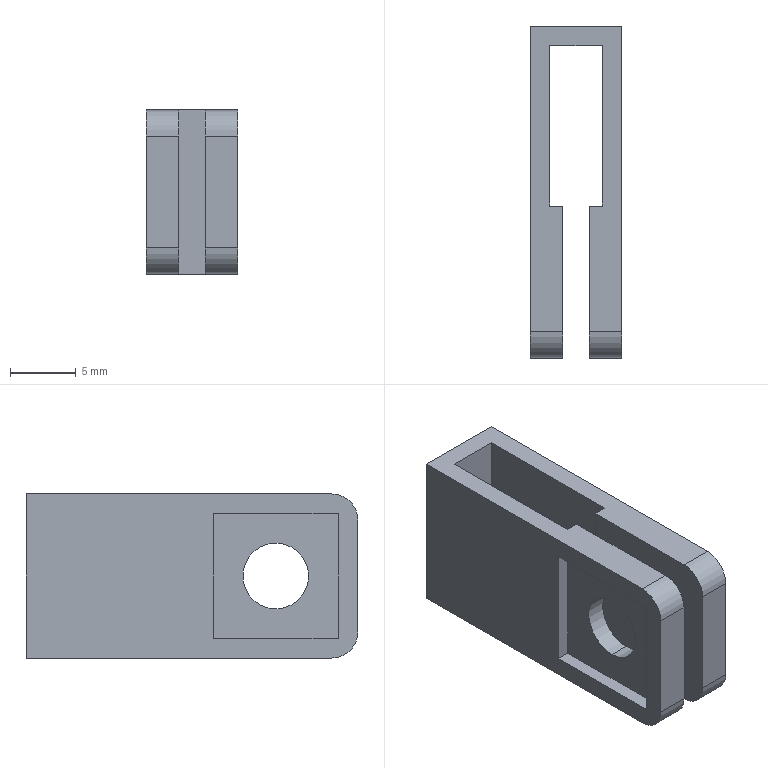Component | SolidWorks | GroundingSystem-1_CopperBarFixingClamp-1 | 1 solid | 32 faces | box 7 x 25.25 x 12.5 mm | volume 1063 mm3 | plane 24 | cylinder 8 | commonest cylinder face diameters 5 x4 4 x4
STEP:
#1=COLOUR_RGB('',0.7922,0.8196,0.9333);
#2=FILL_AREA_STYLE_COLOUR('',#1);
#3=FILL_AREA_STYLE('',(#2));
#4=SURFACE_STYLE_FILL_AREA(#3);
#5=SURFACE_SIDE_STYLE('',(#4));
#6=SURFACE_STYLE_USAGE(.BOTH.,#5);
#7=PRESENTATION_STYLE_ASSIGNMENT((#6));
#8=CARTESIAN_POINT('',(10.466,-0.8639,55.742));
#9=VERTEX_POINT('',#8);
#10=CARTESIAN_POINT('',(10.466,-0.8639,55.545));
#11=VERTEX_POINT('',#10);
#12=CARTESIAN_POINT('',(10.466,-0.8639,55.643));
#13=DIRECTION('',(-1.,0.,0.));
#14=DIRECTION('',(0.,-1.,0.));
#15=AXIS2_PLACEMENT_3D('',#12,#13,#14);
#16=CIRCLE('',#15,0.09843);
#17=EDGE_CURVE('',#9,#11,#16,.T.);
#18=ORIENTED_EDGE('',*,*,#17,.T.);
#19=CARTESIAN_POINT('',(10.525,-0.8639,55.545));
#20=VERTEX_POINT('',#19);
#21=CARTESIAN_POINT('',(10.289,-0.8639,55.545));
#22=DIRECTION('',(1.,-0.,-0.));
#23=VECTOR('',#22,39.37);
#24=LINE('',#21,#23);
#25=EDGE_CURVE('',#11,#20,#24,.T.);
#26=ORIENTED_EDGE('',*,*,#25,.T.);
#27=CARTESIAN_POINT('',(10.525,-0.8639,55.742));
#28=VERTEX_POINT('',#27);
#29=CARTESIAN_POINT('',(10.525,-0.8639,55.643));
#30=DIRECTION('',(-1.,0.,0.));
#31=DIRECTION('',(0.,0.,1.));
#32=AXIS2_PLACEMENT_3D('',#29,#30,#31);
#33=CIRCLE('',#32,0.09843);
#34=EDGE_CURVE('',#28,#20,#33,.T.);
#35=ORIENTED_EDGE('',*,*,#34,.F.);
#36=CARTESIAN_POINT('',(10.289,-0.8639,55.742));
#37=DIRECTION('',(1.,-0.,-0.));
#38=VECTOR('',#37,39.37);
#39=LINE('',#36,#38);
#40=EDGE_CURVE('',#9,#28,#39,.T.);
#41=ORIENTED_EDGE('',*,*,#40,.F.);
#42=EDGE_LOOP('',(#18,#26,#35,#41));
#43=FACE_OUTER_BOUND('',#42,.T.);
#44=CARTESIAN_POINT('',(10.289,-0.8639,55.643));
#45=DIRECTION('',(1.,-0.,-0.));
#46=DIRECTION('',(0.,0.,1.));
#47=AXIS2_PLACEMENT_3D('',#44,#45,#46);
#48=CYLINDRICAL_SURFACE('',#47,0.09843);
#49=ADVANCED_FACE('',(#43),#48,.F.);
#50=CARTESIAN_POINT('',(10.328,-0.8639,55.545));
#51=VERTEX_POINT('',#50);
#52=CARTESIAN_POINT('',(10.328,-0.8639,55.742));
#53=VERTEX_POINT('',#52);
#54=CARTESIAN_POINT('',(10.328,-0.8639,55.643));
#55=DIRECTION('',(1.,-0.,-0.));
#56=DIRECTION('',(0.,-0.,-1.));
#57=AXIS2_PLACEMENT_3D('',#54,#55,#56);
#58=CIRCLE('',#57,0.09843);
#59=EDGE_CURVE('',#51,#53,#58,.T.);
#60=ORIENTED_EDGE('',*,*,#59,.F.);
#61=CARTESIAN_POINT('',(10.387,-0.8639,55.545));
#62=VERTEX_POINT('',#61);
#63=CARTESIAN_POINT('',(10.289,-0.8639,55.545));
#64=DIRECTION('',(1.,-0.,-0.));
#65=VECTOR('',#64,39.37);
#66=LINE('',#63,#65);
#67=EDGE_CURVE('',#51,#62,#66,.T.);
#68=ORIENTED_EDGE('',*,*,#67,.T.);
#69=CARTESIAN_POINT('',(10.387,-0.8639,55.742));
#70=VERTEX_POINT('',#69);
#71=CARTESIAN_POINT('',(10.387,-0.8639,55.643));
#72=DIRECTION('',(1.,0.,-0.));
#73=DIRECTION('',(0.,1.,0.));
#74=AXIS2_PLACEMENT_3D('',#71,#72,#73);
#75=CIRCLE('',#74,0.09843);
#76=EDGE_CURVE('',#62,#70,#75,.T.);
#77=ORIENTED_EDGE('',*,*,#76,.T.);
#78=CARTESIAN_POINT('',(10.289,-0.8639,55.742));
#79=DIRECTION('',(1.,-0.,-0.));
#80=VECTOR('',#79,39.37);
#81=LINE('',#78,#80);
#82=EDGE_CURVE('',#53,#70,#81,.T.);
#83=ORIENTED_EDGE('',*,*,#82,.F.);
#84=EDGE_LOOP('',(#60,#68,#77,#83));
#85=FACE_OUTER_BOUND('',#84,.T.);
#86=CARTESIAN_POINT('',(10.289,-0.8639,55.643));
#87=DIRECTION('',(1.,-0.,-0.));
#88=DIRECTION('',(0.,0.,1.));
#89=AXIS2_PLACEMENT_3D('',#86,#87,#88);
#90=CYLINDRICAL_SURFACE('',#89,0.09843);
#91=ADVANCED_FACE('',(#85),#90,.F.);
#92=CARTESIAN_POINT('',(10.289,-0.1159,55.397));
#93=VERTEX_POINT('',#92);
#94=CARTESIAN_POINT('',(10.289,-1.031,55.397));
#95=VERTEX_POINT('',#94);
#96=CARTESIAN_POINT('',(10.289,-0.1159,55.397));
#97=DIRECTION('',(-0.,-1.,0.));
#98=VECTOR('',#97,39.37);
#99=LINE('',#96,#98);
#100=EDGE_CURVE('',#93,#95,#99,.T.);
#101=ORIENTED_EDGE('',*,*,#100,.T.);
#102=CARTESIAN_POINT('',(10.289,-1.11,55.476));
#103=VERTEX_POINT('',#102);
#104=CARTESIAN_POINT('',(10.289,-1.031,55.476));
#105=DIRECTION('',(-1.,0.,0.));
#106=DIRECTION('',(0.,-0.,-1.));
#107=AXIS2_PLACEMENT_3D('',#104,#105,#106);
#108=CIRCLE('',#107,0.07874);
#109=EDGE_CURVE('',#95,#103,#108,.T.);
#110=ORIENTED_EDGE('',*,*,#109,.T.);
#111=CARTESIAN_POINT('',(10.289,-1.11,55.811));
#112=VERTEX_POINT('',#111);
#113=CARTESIAN_POINT('',(10.289,-1.11,55.397));
#114=DIRECTION('',(0.,0.,1.));
#115=VECTOR('',#114,39.37);
#116=LINE('',#113,#115);
#117=EDGE_CURVE('',#103,#112,#116,.T.);
#118=ORIENTED_EDGE('',*,*,#117,.T.);
#119=CARTESIAN_POINT('',(10.289,-1.031,55.889));
#120=VERTEX_POINT('',#119);
#121=CARTESIAN_POINT('',(10.289,-1.031,55.811));
#122=DIRECTION('',(-1.,0.,0.));
#123=DIRECTION('',(0.,-0.,-1.));
#124=AXIS2_PLACEMENT_3D('',#121,#122,#123);
#125=CIRCLE('',#124,0.07874);
#126=EDGE_CURVE('',#112,#120,#125,.T.);
#127=ORIENTED_EDGE('',*,*,#126,.T.);
#128=CARTESIAN_POINT('',(10.289,-0.1159,55.889));
#129=VERTEX_POINT('',#128);
#130=CARTESIAN_POINT('',(10.289,-0.1159,55.889));
#131=DIRECTION('',(-0.,-1.,0.));
#132=VECTOR('',#131,39.37);
#133=LINE('',#130,#132);
#134=EDGE_CURVE('',#129,#120,#133,.T.);
#135=ORIENTED_EDGE('',*,*,#134,.F.);
#136=CARTESIAN_POINT('',(10.289,-0.1159,55.397));
#137=DIRECTION('',(0.,0.,1.));
#138=VECTOR('',#137,39.37);
#139=LINE('',#136,#138);
#140=EDGE_CURVE('',#93,#129,#139,.T.);
#141=ORIENTED_EDGE('',*,*,#140,.F.);
#142=EDGE_LOOP('',(#101,#110,#118,#127,#135,#141));
#143=FACE_OUTER_BOUND('',#142,.T.);
#144=CARTESIAN_POINT('',(10.289,-0.6769,55.83));
#145=VERTEX_POINT('',#144);
#146=CARTESIAN_POINT('',(10.289,-1.051,55.83));
#147=VERTEX_POINT('',#146);
#148=CARTESIAN_POINT('',(10.289,-0.6769,55.83));
#149=DIRECTION('',(-0.,-1.,0.));
#150=VECTOR('',#149,39.37);
#151=LINE('',#148,#150);
#152=EDGE_CURVE('',#145,#147,#151,.T.);
#153=ORIENTED_EDGE('',*,*,#152,.T.);
#154=CARTESIAN_POINT('',(10.289,-1.051,55.456));
#155=VERTEX_POINT('',#154);
#156=CARTESIAN_POINT('',(10.289,-1.051,55.83));
#157=DIRECTION('',(-0.,-0.,-1.));
#158=VECTOR('',#157,39.37);
#159=LINE('',#156,#158);
#160=EDGE_CURVE('',#147,#155,#159,.T.);
#161=ORIENTED_EDGE('',*,*,#160,.T.);
#162=CARTESIAN_POINT('',(10.289,-0.6769,55.456));
#163=VERTEX_POINT('',#162);
#164=CARTESIAN_POINT('',(10.289,-1.051,55.456));
#165=DIRECTION('',(0.,1.,-0.));
#166=VECTOR('',#165,39.37);
#167=LINE('',#164,#166);
#168=EDGE_CURVE('',#155,#163,#167,.T.);
#169=ORIENTED_EDGE('',*,*,#168,.T.);
#170=CARTESIAN_POINT('',(10.289,-0.6769,55.456));
#171=DIRECTION('',(0.,0.,1.));
#172=VECTOR('',#171,39.37);
#173=LINE('',#170,#172);
#174=EDGE_CURVE('',#163,#145,#173,.T.);
#175=ORIENTED_EDGE('',*,*,#174,.T.);
#176=EDGE_LOOP('',(#153,#161,#169,#175));
#177=FACE_BOUND('',#176,.T.);
#178=CARTESIAN_POINT('',(10.289,-0.1159,55.397));
#179=DIRECTION('',(-1.,0.,0.));
#180=DIRECTION('',(-0.,-0.,-1.));
#181=AXIS2_PLACEMENT_3D('',#178,#179,#180);
#182=PLANE('',#181);
#183=ADVANCED_FACE('',(#143,#177),#182,.T.);
#184=ORIENTED_EDGE('',*,*,#67,.F.);
#185=CARTESIAN_POINT('',(10.328,-0.8639,55.643));
#186=DIRECTION('',(1.,-0.,-0.));
#187=DIRECTION('',(0.,-0.,-1.));
#188=AXIS2_PLACEMENT_3D('',#185,#186,#187);
#189=CIRCLE('',#188,0.09843);
#190=EDGE_CURVE('',#53,#51,#189,.T.);
#191=ORIENTED_EDGE('',*,*,#190,.F.);
#192=ORIENTED_EDGE('',*,*,#82,.T.);
#193=CARTESIAN_POINT('',(10.387,-0.8639,55.643));
#194=DIRECTION('',(1.,0.,-0.));
#195=DIRECTION('',(0.,1.,0.));
#196=AXIS2_PLACEMENT_3D('',#193,#194,#195);
#197=CIRCLE('',#196,0.09843);
#198=EDGE_CURVE('',#70,#62,#197,.T.);
#199=ORIENTED_EDGE('',*,*,#198,.T.);
#200=EDGE_LOOP('',(#184,#191,#192,#199));
#201=FACE_OUTER_BOUND('',#200,.T.);
#202=CARTESIAN_POINT('',(10.289,-0.8639,55.643));
#203=DIRECTION('',(1.,-0.,-0.));
#204=DIRECTION('',(0.,0.,1.));
#205=AXIS2_PLACEMENT_3D('',#202,#203,#204);
#206=CYLINDRICAL_SURFACE('',#205,0.09843);
#207=ADVANCED_FACE('',(#201),#206,.F.);
#208=ORIENTED_EDGE('',*,*,#25,.F.);
#209=CARTESIAN_POINT('',(10.466,-0.8639,55.643));
#210=DIRECTION('',(-1.,0.,0.));
#211=DIRECTION('',(0.,-1.,0.));
#212=AXIS2_PLACEMENT_3D('',#209,#210,#211);
#213=CIRCLE('',#212,0.09843);
#214=EDGE_CURVE('',#11,#9,#213,.T.);
#215=ORIENTED_EDGE('',*,*,#214,.T.);
#216=ORIENTED_EDGE('',*,*,#40,.T.);
#217=CARTESIAN_POINT('',(10.525,-0.8639,55.643));
#218=DIRECTION('',(-1.,0.,0.));
#219=DIRECTION('',(0.,0.,1.));
#220=AXIS2_PLACEMENT_3D('',#217,#218,#219);
#221=CIRCLE('',#220,0.09843);
#222=EDGE_CURVE('',#20,#28,#221,.T.);
#223=ORIENTED_EDGE('',*,*,#222,.F.);
#224=EDGE_LOOP('',(#208,#215,#216,#223));
#225=FACE_OUTER_BOUND('',#224,.T.);
#226=CARTESIAN_POINT('',(10.289,-0.8639,55.643));
#227=DIRECTION('',(1.,-0.,-0.));
#228=DIRECTION('',(0.,0.,1.));
#229=AXIS2_PLACEMENT_3D('',#226,#227,#228);
#230=CYLINDRICAL_SURFACE('',#229,0.09843);
#231=ADVANCED_FACE('',(#225),#230,.F.);
#232=CARTESIAN_POINT('',(10.466,-1.11,55.811));
#233=VERTEX_POINT('',#232);
#234=CARTESIAN_POINT('',(10.466,-1.11,55.476));
#235=VERTEX_POINT('',#234);
#236=CARTESIAN_POINT('',(10.466,-1.11,55.397));
#237=DIRECTION('',(-0.,-0.,-1.));
#238=VECTOR('',#237,39.37);
#239=LINE('',#236,#238);
#240=EDGE_CURVE('',#233,#235,#239,.T.);
#241=ORIENTED_EDGE('',*,*,#240,.T.);
#242=CARTESIAN_POINT('',(10.564,-1.11,55.476));
#243=VERTEX_POINT('',#242);
#244=CARTESIAN_POINT('',(10.289,-1.11,55.476));
#245=DIRECTION('',(1.,-0.,-0.));
#246=VECTOR('',#245,39.37);
#247=LINE('',#244,#246);
#248=EDGE_CURVE('',#235,#243,#247,.T.);
#249=ORIENTED_EDGE('',*,*,#248,.T.);
#250=CARTESIAN_POINT('',(10.564,-1.11,55.811));
#251=VERTEX_POINT('',#250);
#252=CARTESIAN_POINT('',(10.564,-1.11,55.397));
#253=DIRECTION('',(0.,0.,1.));
#254=VECTOR('',#253,39.37);
#255=LINE('',#252,#254);
#256=EDGE_CURVE('',#243,#251,#255,.T.);
#257=ORIENTED_EDGE('',*,*,#256,.T.);
#258=CARTESIAN_POINT('',(10.466,-1.11,55.811));
#259=DIRECTION('',(-1.,0.,0.));
#260=VECTOR('',#259,39.37);
#261=LINE('',#258,#260);
#262=EDGE_CURVE('',#251,#233,#261,.T.);
#263=ORIENTED_EDGE('',*,*,#262,.T.);
#264=EDGE_LOOP('',(#241,#249,#257,#263));
#265=FACE_OUTER_BOUND('',#264,.T.);
#266=CARTESIAN_POINT('',(10.289,-1.11,55.397));
#267=DIRECTION('',(-0.,-1.,0.));
#268=DIRECTION('',(-0.,-0.,-1.));
#269=AXIS2_PLACEMENT_3D('',#266,#267,#268);
#270=PLANE('',#269);
#271=ADVANCED_FACE('',(#265),#270,.T.);
#272=ORIENTED_EDGE('',*,*,#117,.F.);
#273=CARTESIAN_POINT('',(10.387,-1.11,55.476));
#274=VERTEX_POINT('',#273);
#275=CARTESIAN_POINT('',(10.289,-1.11,55.476));
#276=DIRECTION('',(1.,-0.,-0.));
#277=VECTOR('',#276,39.37);
#278=LINE('',#275,#277);
#279=EDGE_CURVE('',#103,#274,#278,.T.);
#280=ORIENTED_EDGE('',*,*,#279,.T.);
#281=CARTESIAN_POINT('',(10.387,-1.11,55.811));
#282=VERTEX_POINT('',#281);
#283=CARTESIAN_POINT('',(10.387,-1.11,55.397));
#284=DIRECTION('',(0.,0.,1.));
#285=VECTOR('',#284,39.37);
#286=LINE('',#283,#285);
#287=EDGE_CURVE('',#274,#282,#286,.T.);
#288=ORIENTED_EDGE('',*,*,#287,.T.);
#289=CARTESIAN_POINT('',(10.289,-1.11,55.811));
#290=DIRECTION('',(-1.,0.,0.));
#291=VECTOR('',#290,39.37);
#292=LINE('',#289,#291);
#293=EDGE_CURVE('',#282,#112,#292,.T.);
#294=ORIENTED_EDGE('',*,*,#293,.T.);
#295=EDGE_LOOP('',(#272,#280,#288,#294));
#296=FACE_OUTER_BOUND('',#295,.T.);
#297=CARTESIAN_POINT('',(10.289,-1.11,55.397));
#298=DIRECTION('',(-0.,-1.,0.));
#299=DIRECTION('',(-0.,-0.,-1.));
#300=AXIS2_PLACEMENT_3D('',#297,#298,#299);
#301=PLANE('',#300);
#302=ADVANCED_FACE('',(#296),#301,.T.);
#303=CARTESIAN_POINT('',(10.387,-0.6553,55.397));
#304=VERTEX_POINT('',#303);
#305=CARTESIAN_POINT('',(10.387,-1.031,55.397));
#306=VERTEX_POINT('',#305);
#307=CARTESIAN_POINT('',(10.387,-1.11,55.397));
#308=DIRECTION('',(0.,-1.,0.));
#309=VECTOR('',#308,39.37);
#310=LINE('',#307,#309);
#311=EDGE_CURVE('',#304,#306,#310,.T.);
#312=ORIENTED_EDGE('',*,*,#311,.T.);
#313=CARTESIAN_POINT('',(10.564,-1.031,55.397));
#314=DIRECTION('',(-1.,0.,0.));
#315=VECTOR('',#314,39.37);
#316=LINE('',#313,#315);
#317=EDGE_CURVE('',#306,#95,#316,.T.);
#318=ORIENTED_EDGE('',*,*,#317,.T.);
#319=ORIENTED_EDGE('',*,*,#100,.F.);
#320=CARTESIAN_POINT('',(10.564,-0.1159,55.397));
#321=VERTEX_POINT('',#320);
#322=CARTESIAN_POINT('',(10.289,-0.1159,55.397));
#323=DIRECTION('',(-1.,0.,0.));
#324=VECTOR('',#323,39.37);
#325=LINE('',#322,#324);
#326=EDGE_CURVE('',#321,#93,#325,.T.);
#327=ORIENTED_EDGE('',*,*,#326,.F.);
#328=CARTESIAN_POINT('',(10.564,-1.031,55.397));
#329=VERTEX_POINT('',#328);
#330=CARTESIAN_POINT('',(10.564,-0.1159,55.397));
#331=DIRECTION('',(0.,1.,-0.));
#332=VECTOR('',#331,39.37);
#333=LINE('',#330,#332);
#334=EDGE_CURVE('',#329,#321,#333,.T.);
#335=ORIENTED_EDGE('',*,*,#334,.F.);
#336=CARTESIAN_POINT('',(10.466,-1.031,55.397));
#337=VERTEX_POINT('',#336);
#338=CARTESIAN_POINT('',(10.564,-1.031,55.397));
#339=DIRECTION('',(-1.,0.,0.));
#340=VECTOR('',#339,39.37);
#341=LINE('',#338,#340);
#342=EDGE_CURVE('',#329,#337,#341,.T.);
#343=ORIENTED_EDGE('',*,*,#342,.T.);
#344=CARTESIAN_POINT('',(10.466,-0.6553,55.397));
#345=VERTEX_POINT('',#344);
#346=CARTESIAN_POINT('',(10.466,-1.11,55.397));
#347=DIRECTION('',(0.,1.,-0.));
#348=VECTOR('',#347,39.37);
#349=LINE('',#346,#348);
#350=EDGE_CURVE('',#337,#345,#349,.T.);
#351=ORIENTED_EDGE('',*,*,#350,.T.);
#352=CARTESIAN_POINT('',(10.505,-0.6553,55.397));
#353=VERTEX_POINT('',#352);
#354=CARTESIAN_POINT('',(10.564,-0.6553,55.397));
#355=DIRECTION('',(1.,-0.,-0.));
#356=VECTOR('',#355,39.37);
#357=LINE('',#354,#356);
#358=EDGE_CURVE('',#345,#353,#357,.T.);
#359=ORIENTED_EDGE('',*,*,#358,.T.);
#360=CARTESIAN_POINT('',(10.505,-0.175,55.397));
#361=VERTEX_POINT('',#360);
#362=CARTESIAN_POINT('',(10.505,-1.11,55.397));
#363=DIRECTION('',(0.,1.,-0.));
#364=VECTOR('',#363,39.37);
#365=LINE('',#362,#364);
#366=EDGE_CURVE('',#353,#361,#365,.T.);
#367=ORIENTED_EDGE('',*,*,#366,.T.);
#368=CARTESIAN_POINT('',(10.348,-0.175,55.397));
#369=VERTEX_POINT('',#368);
#370=CARTESIAN_POINT('',(10.564,-0.175,55.397));
#371=DIRECTION('',(-1.,0.,0.));
#372=VECTOR('',#371,39.37);
#373=LINE('',#370,#372);
#374=EDGE_CURVE('',#361,#369,#373,.T.);
#375=ORIENTED_EDGE('',*,*,#374,.T.);
#376=CARTESIAN_POINT('',(10.348,-0.6553,55.397));
#377=VERTEX_POINT('',#376);
#378=CARTESIAN_POINT('',(10.348,-1.11,55.397));
#379=DIRECTION('',(0.,-1.,0.));
#380=VECTOR('',#379,39.37);
#381=LINE('',#378,#380);
#382=EDGE_CURVE('',#369,#377,#381,.T.);
#383=ORIENTED_EDGE('',*,*,#382,.T.);
#384=CARTESIAN_POINT('',(10.564,-0.6553,55.397));
#385=DIRECTION('',(1.,0.,-0.));
#386=VECTOR('',#385,39.37);
#387=LINE('',#384,#386);
#388=EDGE_CURVE('',#377,#304,#387,.T.);
#389=ORIENTED_EDGE('',*,*,#388,.T.);
#390=EDGE_LOOP('',(#312,#318,#319,#327,#335,#343,#351,#359,#367,#375,#383,#389));
#391=FACE_OUTER_BOUND('',#390,.T.);
#392=CARTESIAN_POINT('',(10.564,-1.11,55.397));
#393=DIRECTION('',(-0.,-0.,-1.));
#394=DIRECTION('',(0.,1.,-0.));
#395=AXIS2_PLACEMENT_3D('',#392,#393,#394);
#396=PLANE('',#395);
#397=ADVANCED_FACE('',(#391),#396,.T.);
#398=CARTESIAN_POINT('',(10.466,-1.031,55.889));
#399=VERTEX_POINT('',#398);
#400=CARTESIAN_POINT('',(10.466,-0.6553,55.889));
#401=VERTEX_POINT('',#400);
#402=CARTESIAN_POINT('',(10.466,-1.11,55.889));
#403=DIRECTION('',(0.,1.,-0.));
#404=VECTOR('',#403,39.37);
#405=LINE('',#402,#404);
#406=EDGE_CURVE('',#399,#401,#405,.T.);
#407=ORIENTED_EDGE('',*,*,#406,.F.);
#408=CARTESIAN_POINT('',(10.564,-1.031,55.889));
#409=VERTEX_POINT('',#408);
#410=CARTESIAN_POINT('',(10.564,-1.031,55.889));
#411=DIRECTION('',(1.,-0.,-0.));
#412=VECTOR('',#411,39.37);
#413=LINE('',#410,#412);
#414=EDGE_CURVE('',#399,#409,#413,.T.);
#415=ORIENTED_EDGE('',*,*,#414,.T.);
#416=CARTESIAN_POINT('',(10.564,-0.1159,55.889));
#417=VERTEX_POINT('',#416);
#418=CARTESIAN_POINT('',(10.564,-0.1159,55.889));
#419=DIRECTION('',(0.,1.,-0.));
#420=VECTOR('',#419,39.37);
#421=LINE('',#418,#420);
#422=EDGE_CURVE('',#409,#417,#421,.T.);
#423=ORIENTED_EDGE('',*,*,#422,.T.);
#424=CARTESIAN_POINT('',(10.289,-0.1159,55.889));
#425=DIRECTION('',(-1.,0.,0.));
#426=VECTOR('',#425,39.37);
#427=LINE('',#424,#426);
#428=EDGE_CURVE('',#417,#129,#427,.T.);
#429=ORIENTED_EDGE('',*,*,#428,.T.);
#430=ORIENTED_EDGE('',*,*,#134,.T.);
#431=CARTESIAN_POINT('',(10.387,-1.031,55.889));
#432=VERTEX_POINT('',#431);
#433=CARTESIAN_POINT('',(10.387,-1.031,55.889));
#434=DIRECTION('',(1.,-0.,-0.));
#435=VECTOR('',#434,39.37);
#436=LINE('',#433,#435);
#437=EDGE_CURVE('',#120,#432,#436,.T.);
#438=ORIENTED_EDGE('',*,*,#437,.T.);
#439=CARTESIAN_POINT('',(10.387,-0.6553,55.889));
#440=VERTEX_POINT('',#439);
#441=CARTESIAN_POINT('',(10.387,-1.11,55.889));
#442=DIRECTION('',(0.,-1.,0.));
#443=VECTOR('',#442,39.37);
#444=LINE('',#441,#443);
#445=EDGE_CURVE('',#440,#432,#444,.T.);
#446=ORIENTED_EDGE('',*,*,#445,.F.);
#447=CARTESIAN_POINT('',(10.348,-0.6553,55.889));
#448=VERTEX_POINT('',#447);
#449=CARTESIAN_POINT('',(10.564,-0.6553,55.889));
#450=DIRECTION('',(1.,0.,-0.));
#451=VECTOR('',#450,39.37);
#452=LINE('',#449,#451);
#453=EDGE_CURVE('',#448,#440,#452,.T.);
#454=ORIENTED_EDGE('',*,*,#453,.F.);
#455=CARTESIAN_POINT('',(10.348,-0.175,55.889));
#456=VERTEX_POINT('',#455);
#457=CARTESIAN_POINT('',(10.348,-1.11,55.889));
#458=DIRECTION('',(0.,-1.,0.));
#459=VECTOR('',#458,39.37);
#460=LINE('',#457,#459);
#461=EDGE_CURVE('',#456,#448,#460,.T.);
#462=ORIENTED_EDGE('',*,*,#461,.F.);
#463=CARTESIAN_POINT('',(10.505,-0.175,55.889));
#464=VERTEX_POINT('',#463);
#465=CARTESIAN_POINT('',(10.564,-0.175,55.889));
#466=DIRECTION('',(-1.,0.,0.));
#467=VECTOR('',#466,39.37);
#468=LINE('',#465,#467);
#469=EDGE_CURVE('',#464,#456,#468,.T.);
#470=ORIENTED_EDGE('',*,*,#469,.F.);
#471=CARTESIAN_POINT('',(10.505,-0.6553,55.889));
#472=VERTEX_POINT('',#471);
#473=CARTESIAN_POINT('',(10.505,-1.11,55.889));
#474=DIRECTION('',(0.,1.,-0.));
#475=VECTOR('',#474,39.37);
#476=LINE('',#473,#475);
#477=EDGE_CURVE('',#472,#464,#476,.T.);
#478=ORIENTED_EDGE('',*,*,#477,.F.);
#479=CARTESIAN_POINT('',(10.564,-0.6553,55.889));
#480=DIRECTION('',(1.,-0.,-0.));
#481=VECTOR('',#480,39.37);
#482=LINE('',#479,#481);
#483=EDGE_CURVE('',#401,#472,#482,.T.);
#484=ORIENTED_EDGE('',*,*,#483,.F.);
#485=EDGE_LOOP('',(#407,#415,#423,#429,#430,#438,#446,#454,#462,#470,#478,#484));
#486=FACE_OUTER_BOUND('',#485,.T.);
#487=CARTESIAN_POINT('',(10.564,-1.11,55.889));
#488=DIRECTION('',(-0.,-0.,-1.));
#489=DIRECTION('',(0.,1.,-0.));
#490=AXIS2_PLACEMENT_3D('',#487,#488,#489);
#491=PLANE('',#490);
#492=ADVANCED_FACE('',(#486),#491,.F.);
#493=ORIENTED_EDGE('',*,*,#428,.F.);
#494=CARTESIAN_POINT('',(10.564,-0.1159,55.397));
#495=DIRECTION('',(0.,0.,1.));
#496=VECTOR('',#495,39.37);
#497=LINE('',#494,#496);
#498=EDGE_CURVE('',#321,#417,#497,.T.);
#499=ORIENTED_EDGE('',*,*,#498,.F.);
#500=ORIENTED_EDGE('',*,*,#326,.T.);
#501=ORIENTED_EDGE('',*,*,#140,.T.);
#502=EDGE_LOOP('',(#493,#499,#500,#501));
#503=FACE_OUTER_BOUND('',#502,.T.);
#504=CARTESIAN_POINT('',(10.289,-0.1159,55.397));
#505=DIRECTION('',(0.,1.,-0.));
#506=DIRECTION('',(0.,0.,1.));
#507=AXIS2_PLACEMENT_3D('',#504,#505,#506);
#508=PLANE('',#507);
#509=ADVANCED_FACE('',(#503),#508,.T.);
#510=CARTESIAN_POINT('',(10.564,-1.051,55.83));
#511=VERTEX_POINT('',#510);
#512=CARTESIAN_POINT('',(10.564,-1.051,55.456));
#513=VERTEX_POINT('',#512);
#514=CARTESIAN_POINT('',(10.564,-1.051,55.83));
#515=DIRECTION('',(-0.,-0.,-1.));
#516=VECTOR('',#515,39.37);
#517=LINE('',#514,#516);
#518=EDGE_CURVE('',#511,#513,#517,.T.);
#519=ORIENTED_EDGE('',*,*,#518,.F.);
#520=CARTESIAN_POINT('',(10.564,-0.6769,55.83));
#521=VERTEX_POINT('',#520);
#522=CARTESIAN_POINT('',(10.564,-0.6769,55.83));
#523=DIRECTION('',(-0.,-1.,0.));
#524=VECTOR('',#523,39.37);
#525=LINE('',#522,#524);
#526=EDGE_CURVE('',#521,#511,#525,.T.);
#527=ORIENTED_EDGE('',*,*,#526,.F.);
#528=CARTESIAN_POINT('',(10.564,-0.6769,55.456));
#529=VERTEX_POINT('',#528);
#530=CARTESIAN_POINT('',(10.564,-0.6769,55.456));
#531=DIRECTION('',(0.,0.,1.));
#532=VECTOR('',#531,39.37);
#533=LINE('',#530,#532);
#534=EDGE_CURVE('',#529,#521,#533,.T.);
#535=ORIENTED_EDGE('',*,*,#534,.F.);
#536=CARTESIAN_POINT('',(10.564,-1.051,55.456));
#537=DIRECTION('',(0.,1.,-0.));
#538=VECTOR('',#537,39.37);
#539=LINE('',#536,#538);
#540=EDGE_CURVE('',#513,#529,#539,.T.);
#541=ORIENTED_EDGE('',*,*,#540,.F.);
#542=EDGE_LOOP('',(#519,#527,#535,#541));
#543=FACE_BOUND('',#542,.T.);
#544=ORIENTED_EDGE('',*,*,#256,.F.);
#545=CARTESIAN_POINT('',(10.564,-1.031,55.476));
#546=DIRECTION('',(1.,-0.,-0.));
#547=DIRECTION('',(0.,0.,1.));
#548=AXIS2_PLACEMENT_3D('',#545,#546,#547);
#549=CIRCLE('',#548,0.07874);
#550=EDGE_CURVE('',#243,#329,#549,.T.);
#551=ORIENTED_EDGE('',*,*,#550,.T.);
#552=ORIENTED_EDGE('',*,*,#334,.T.);
#553=ORIENTED_EDGE('',*,*,#498,.T.);
#554=ORIENTED_EDGE('',*,*,#422,.F.);
#555=CARTESIAN_POINT('',(10.564,-1.031,55.811));
#556=DIRECTION('',(1.,-0.,-0.));
#557=DIRECTION('',(0.,0.,1.));
#558=AXIS2_PLACEMENT_3D('',#555,#556,#557);
#559=CIRCLE('',#558,0.07874);
#560=EDGE_CURVE('',#409,#251,#559,.T.);
#561=ORIENTED_EDGE('',*,*,#560,.T.);
#562=EDGE_LOOP('',(#544,#551,#552,#553,#554,#561));
#563=FACE_OUTER_BOUND('',#562,.T.);
#564=CARTESIAN_POINT('',(10.564,-0.1159,55.397));
#565=DIRECTION('',(1.,-0.,-0.));
#566=DIRECTION('',(0.,0.,1.));
#567=AXIS2_PLACEMENT_3D('',#564,#565,#566);
#568=PLANE('',#567);
#569=ADVANCED_FACE('',(#543,#563),#568,.T.);
#570=ORIENTED_EDGE('',*,*,#358,.F.);
#571=CARTESIAN_POINT('',(10.466,-0.6553,57.318));
#572=DIRECTION('',(-0.,-0.,-1.));
#573=VECTOR('',#572,39.37);
#574=LINE('',#571,#573);
#575=EDGE_CURVE('',#401,#345,#574,.T.);
#576=ORIENTED_EDGE('',*,*,#575,.F.);
#577=ORIENTED_EDGE('',*,*,#483,.T.);
#578=CARTESIAN_POINT('',(10.505,-0.6553,57.318));
#579=DIRECTION('',(-0.,-0.,-1.));
#580=VECTOR('',#579,39.37);
#581=LINE('',#578,#580);
#582=EDGE_CURVE('',#472,#353,#581,.T.);
#583=ORIENTED_EDGE('',*,*,#582,.T.);
#584=EDGE_LOOP('',(#570,#576,#577,#583));
#585=FACE_OUTER_BOUND('',#584,.T.);
#586=CARTESIAN_POINT('',(10.505,-0.6553,57.318));
#587=DIRECTION('',(0.,1.,-0.));
#588=DIRECTION('',(-1.,0.,0.));
#589=AXIS2_PLACEMENT_3D('',#586,#587,#588);
#590=PLANE('',#589);
#591=ADVANCED_FACE('',(#585),#590,.T.);
#592=ORIENTED_EDGE('',*,*,#366,.F.);
#593=ORIENTED_EDGE('',*,*,#582,.F.);
#594=ORIENTED_EDGE('',*,*,#477,.T.);
#595=CARTESIAN_POINT('',(10.505,-0.175,57.318));
#596=DIRECTION('',(-0.,-0.,-1.));
#597=VECTOR('',#596,39.37);
#598=LINE('',#595,#597);
#599=EDGE_CURVE('',#464,#361,#598,.T.);
#600=ORIENTED_EDGE('',*,*,#599,.T.);
#601=EDGE_LOOP('',(#592,#593,#594,#600));
#602=FACE_OUTER_BOUND('',#601,.T.);
#603=CARTESIAN_POINT('',(10.505,-0.175,57.318));
#604=DIRECTION('',(-1.,0.,0.));
#605=DIRECTION('',(-0.,-1.,0.));
#606=AXIS2_PLACEMENT_3D('',#603,#604,#605);
#607=PLANE('',#606);
#608=ADVANCED_FACE('',(#602),#607,.T.);
#609=ORIENTED_EDGE('',*,*,#374,.F.);
#610=ORIENTED_EDGE('',*,*,#599,.F.);
#611=ORIENTED_EDGE('',*,*,#469,.T.);
#612=CARTESIAN_POINT('',(10.348,-0.175,57.318));
#613=DIRECTION('',(-0.,-0.,-1.));
#614=VECTOR('',#613,39.37);
#615=LINE('',#612,#614);
#616=EDGE_CURVE('',#456,#369,#615,.T.);
#617=ORIENTED_EDGE('',*,*,#616,.T.);
#618=EDGE_LOOP('',(#609,#610,#611,#617));
#619=FACE_OUTER_BOUND('',#618,.T.);
#620=CARTESIAN_POINT('',(10.348,-0.175,57.318));
#621=DIRECTION('',(-0.,-1.,0.));
#622=DIRECTION('',(-0.,-0.,-1.));
#623=AXIS2_PLACEMENT_3D('',#620,#621,#622);
#624=PLANE('',#623);
#625=ADVANCED_FACE('',(#619),#624,.T.);
#626=ORIENTED_EDGE('',*,*,#382,.F.);
#627=ORIENTED_EDGE('',*,*,#616,.F.);
#628=ORIENTED_EDGE('',*,*,#461,.T.);
#629=CARTESIAN_POINT('',(10.348,-0.6553,57.318));
#630=DIRECTION('',(-0.,-0.,-1.));
#631=VECTOR('',#630,39.37);
#632=LINE('',#629,#631);
#633=EDGE_CURVE('',#448,#377,#632,.T.);
#634=ORIENTED_EDGE('',*,*,#633,.T.);
#635=EDGE_LOOP('',(#626,#627,#628,#634));
#636=FACE_OUTER_BOUND('',#635,.T.);
#637=CARTESIAN_POINT('',(10.348,-0.175,57.318));
#638=DIRECTION('',(1.,0.,-0.));
#639=DIRECTION('',(-0.,1.,-0.));
#640=AXIS2_PLACEMENT_3D('',#637,#638,#639);
#641=PLANE('',#640);
#642=ADVANCED_FACE('',(#636),#641,.T.);
#643=ORIENTED_EDGE('',*,*,#388,.F.);
#644=ORIENTED_EDGE('',*,*,#633,.F.);
#645=ORIENTED_EDGE('',*,*,#453,.T.);
#646=CARTESIAN_POINT('',(10.387,-0.6553,57.318));
#647=DIRECTION('',(-0.,-0.,-1.));
#648=VECTOR('',#647,39.37);
#649=LINE('',#646,#648);
#650=EDGE_CURVE('',#440,#304,#649,.T.);
#651=ORIENTED_EDGE('',*,*,#650,.T.);
#652=EDGE_LOOP('',(#643,#644,#645,#651));
#653=FACE_OUTER_BOUND('',#652,.T.);
#654=CARTESIAN_POINT('',(10.348,-0.6553,57.318));
#655=DIRECTION('',(-0.,1.,-0.));
#656=DIRECTION('',(-1.,-0.,0.));
#657=AXIS2_PLACEMENT_3D('',#654,#655,#656);
#658=PLANE('',#657);
#659=ADVANCED_FACE('',(#653),#658,.T.);
#660=ORIENTED_EDGE('',*,*,#17,.F.);
#661=ORIENTED_EDGE('',*,*,#214,.F.);
#662=EDGE_LOOP('',(#660,#661));
#663=FACE_BOUND('',#662,.T.);
#664=ORIENTED_EDGE('',*,*,#350,.F.);
#665=CARTESIAN_POINT('',(10.466,-1.031,55.476));
#666=DIRECTION('',(-1.,0.,0.));
#667=DIRECTION('',(0.,-1.,0.));
#668=AXIS2_PLACEMENT_3D('',#665,#666,#667);
#669=CIRCLE('',#668,0.07874);
#670=EDGE_CURVE('',#337,#235,#669,.T.);
#671=ORIENTED_EDGE('',*,*,#670,.T.);
#672=ORIENTED_EDGE('',*,*,#240,.F.);
#673=CARTESIAN_POINT('',(10.466,-1.031,55.811));
#674=DIRECTION('',(-1.,0.,0.));
#675=DIRECTION('',(0.,-1.,0.));
#676=AXIS2_PLACEMENT_3D('',#673,#674,#675);
#677=CIRCLE('',#676,0.07874);
#678=EDGE_CURVE('',#233,#399,#677,.T.);
#679=ORIENTED_EDGE('',*,*,#678,.T.);
#680=ORIENTED_EDGE('',*,*,#406,.T.);
#681=ORIENTED_EDGE('',*,*,#575,.T.);
#682=EDGE_LOOP('',(#664,#671,#672,#679,#680,#681));
#683=FACE_OUTER_BOUND('',#682,.T.);
#684=CARTESIAN_POINT('',(10.466,-0.6553,57.318));
#685=DIRECTION('',(-1.,0.,0.));
#686=DIRECTION('',(-0.,-1.,0.));
#687=AXIS2_PLACEMENT_3D('',#684,#685,#686);
#688=PLANE('',#687);
#689=ADVANCED_FACE('',(#663,#683),#688,.T.);
#690=ORIENTED_EDGE('',*,*,#198,.F.);
#691=ORIENTED_EDGE('',*,*,#76,.F.);
#692=EDGE_LOOP('',(#690,#691));
#693=FACE_BOUND('',#692,.T.);
#694=ORIENTED_EDGE('',*,*,#287,.F.);
#695=CARTESIAN_POINT('',(10.387,-1.031,55.476));
#696=DIRECTION('',(1.,0.,-0.));
#697=DIRECTION('',(0.,1.,0.));
#698=AXIS2_PLACEMENT_3D('',#695,#696,#697);
#699=CIRCLE('',#698,0.07874);
#700=EDGE_CURVE('',#274,#306,#699,.T.);
#701=ORIENTED_EDGE('',*,*,#700,.T.);
#702=ORIENTED_EDGE('',*,*,#311,.F.);
#703=ORIENTED_EDGE('',*,*,#650,.F.);
#704=ORIENTED_EDGE('',*,*,#445,.T.);
#705=CARTESIAN_POINT('',(10.387,-1.031,55.811));
#706=DIRECTION('',(1.,0.,-0.));
#707=DIRECTION('',(0.,1.,0.));
#708=AXIS2_PLACEMENT_3D('',#705,#706,#707);
#709=CIRCLE('',#708,0.07874);
#710=EDGE_CURVE('',#432,#282,#709,.T.);
#711=ORIENTED_EDGE('',*,*,#710,.T.);
#712=EDGE_LOOP('',(#694,#701,#702,#703,#704,#711));
#713=FACE_OUTER_BOUND('',#712,.T.);
#714=CARTESIAN_POINT('',(10.387,-0.6553,57.318));
#715=DIRECTION('',(1.,0.,-0.));
#716=DIRECTION('',(-0.,1.,-0.));
#717=AXIS2_PLACEMENT_3D('',#714,#715,#716);
#718=PLANE('',#717);
#719=ADVANCED_FACE('',(#693,#713),#718,.T.);
#720=CARTESIAN_POINT('',(10.525,-1.051,55.83));
#721=VERTEX_POINT('',#720);
#722=CARTESIAN_POINT('',(10.525,-1.051,55.456));
#723=VERTEX_POINT('',#722);
#724=CARTESIAN_POINT('',(10.525,-1.051,55.83));
#725=DIRECTION('',(-0.,-0.,-1.));
#726=VECTOR('',#725,39.37);
#727=LINE('',#724,#726);
#728=EDGE_CURVE('',#721,#723,#727,.T.);
#729=ORIENTED_EDGE('',*,*,#728,.T.);
#730=CARTESIAN_POINT('',(10.525,-0.6769,55.456));
#731=VERTEX_POINT('',#730);
#732=CARTESIAN_POINT('',(10.525,-1.051,55.456));
#733=DIRECTION('',(0.,1.,-0.));
#734=VECTOR('',#733,39.37);
#735=LINE('',#732,#734);
#736=EDGE_CURVE('',#723,#731,#735,.T.);
#737=ORIENTED_EDGE('',*,*,#736,.T.);
#738=CARTESIAN_POINT('',(10.525,-0.6769,55.83));
#739=VERTEX_POINT('',#738);
#740=CARTESIAN_POINT('',(10.525,-0.6769,55.456));
#741=DIRECTION('',(0.,0.,1.));
#742=VECTOR('',#741,39.37);
#743=LINE('',#740,#742);
#744=EDGE_CURVE('',#731,#739,#743,.T.);
#745=ORIENTED_EDGE('',*,*,#744,.T.);
#746=CARTESIAN_POINT('',(10.525,-0.6769,55.83));
#747=DIRECTION('',(-0.,-1.,0.));
#748=VECTOR('',#747,39.37);
#749=LINE('',#746,#748);
#750=EDGE_CURVE('',#739,#721,#749,.T.);
#751=ORIENTED_EDGE('',*,*,#750,.T.);
#752=EDGE_LOOP('',(#729,#737,#745,#751));
#753=FACE_OUTER_BOUND('',#752,.T.);
#754=ORIENTED_EDGE('',*,*,#34,.T.);
#755=ORIENTED_EDGE('',*,*,#222,.T.);
#756=EDGE_LOOP('',(#754,#755));
#757=FACE_BOUND('',#756,.T.);
#758=CARTESIAN_POINT('',(10.525,-1.051,55.456));
#759=DIRECTION('',(1.,-0.,-0.));
#760=DIRECTION('',(0.,0.,1.));
#761=AXIS2_PLACEMENT_3D('',#758,#759,#760);
#762=PLANE('',#761);
#763=ADVANCED_FACE('',(#753,#757),#762,.T.);
#764=ORIENTED_EDGE('',*,*,#518,.T.);
#765=CARTESIAN_POINT('',(10.525,-1.051,55.456));
#766=DIRECTION('',(1.,-0.,-0.));
#767=VECTOR('',#766,39.37);
#768=LINE('',#765,#767);
#769=EDGE_CURVE('',#723,#513,#768,.T.);
#770=ORIENTED_EDGE('',*,*,#769,.F.);
#771=ORIENTED_EDGE('',*,*,#728,.F.);
#772=CARTESIAN_POINT('',(10.525,-1.051,55.83));
#773=DIRECTION('',(1.,-0.,-0.));
#774=VECTOR('',#773,39.37);
#775=LINE('',#772,#774);
#776=EDGE_CURVE('',#721,#511,#775,.T.);
#777=ORIENTED_EDGE('',*,*,#776,.T.);
#778=EDGE_LOOP('',(#764,#770,#771,#777));
#779=FACE_OUTER_BOUND('',#778,.T.);
#780=CARTESIAN_POINT('',(10.525,-1.051,55.83));
#781=DIRECTION('',(-0.,-1.,0.));
#782=DIRECTION('',(-0.,-0.,-1.));
#783=AXIS2_PLACEMENT_3D('',#780,#781,#782);
#784=PLANE('',#783);
#785=ADVANCED_FACE('',(#779),#784,.F.);
#786=ORIENTED_EDGE('',*,*,#526,.T.);
#787=ORIENTED_EDGE('',*,*,#776,.F.);
#788=ORIENTED_EDGE('',*,*,#750,.F.);
#789=CARTESIAN_POINT('',(10.525,-0.6769,55.83));
#790=DIRECTION('',(1.,-0.,-0.));
#791=VECTOR('',#790,39.37);
#792=LINE('',#789,#791);
#793=EDGE_CURVE('',#739,#521,#792,.T.);
#794=ORIENTED_EDGE('',*,*,#793,.T.);
#795=EDGE_LOOP('',(#786,#787,#788,#794));
#796=FACE_OUTER_BOUND('',#795,.T.);
#797=CARTESIAN_POINT('',(10.525,-0.6769,55.83));
#798=DIRECTION('',(0.,0.,1.));
#799=DIRECTION('',(-0.,-1.,0.));
#800=AXIS2_PLACEMENT_3D('',#797,#798,#799);
#801=PLANE('',#800);
#802=ADVANCED_FACE('',(#796),#801,.F.);
#803=ORIENTED_EDGE('',*,*,#534,.T.);
#804=ORIENTED_EDGE('',*,*,#793,.F.);
#805=ORIENTED_EDGE('',*,*,#744,.F.);
#806=CARTESIAN_POINT('',(10.525,-0.6769,55.456));
#807=DIRECTION('',(1.,-0.,-0.));
#808=VECTOR('',#807,39.37);
#809=LINE('',#806,#808);
#810=EDGE_CURVE('',#731,#529,#809,.T.);
#811=ORIENTED_EDGE('',*,*,#810,.T.);
#812=EDGE_LOOP('',(#803,#804,#805,#811));
#813=FACE_OUTER_BOUND('',#812,.T.);
#814=CARTESIAN_POINT('',(10.525,-0.6769,55.456));
#815=DIRECTION('',(0.,1.,-0.));
#816=DIRECTION('',(0.,0.,1.));
#817=AXIS2_PLACEMENT_3D('',#814,#815,#816);
#818=PLANE('',#817);
#819=ADVANCED_FACE('',(#813),#818,.F.);
#820=ORIENTED_EDGE('',*,*,#540,.T.);
#821=ORIENTED_EDGE('',*,*,#810,.F.);
#822=ORIENTED_EDGE('',*,*,#736,.F.);
#823=ORIENTED_EDGE('',*,*,#769,.T.);
#824=EDGE_LOOP('',(#820,#821,#822,#823));
#825=FACE_OUTER_BOUND('',#824,.T.);
#826=CARTESIAN_POINT('',(10.525,-1.051,55.456));
#827=DIRECTION('',(-0.,-0.,-1.));
#828=DIRECTION('',(0.,1.,-0.));
#829=AXIS2_PLACEMENT_3D('',#826,#827,#828);
#830=PLANE('',#829);
#831=ADVANCED_FACE('',(#825),#830,.F.);
#832=CARTESIAN_POINT('',(10.328,-1.051,55.83));
#833=VERTEX_POINT('',#832);
#834=CARTESIAN_POINT('',(10.328,-1.051,55.456));
#835=VERTEX_POINT('',#834);
#836=CARTESIAN_POINT('',(10.328,-1.051,55.83));
#837=DIRECTION('',(-0.,-0.,-1.));
#838=VECTOR('',#837,39.37);
#839=LINE('',#836,#838);
#840=EDGE_CURVE('',#833,#835,#839,.T.);
#841=ORIENTED_EDGE('',*,*,#840,.F.);
#842=CARTESIAN_POINT('',(10.328,-0.6769,55.83));
#843=VERTEX_POINT('',#842);
#844=CARTESIAN_POINT('',(10.328,-0.6769,55.83));
#845=DIRECTION('',(-0.,-1.,0.));
#846=VECTOR('',#845,39.37);
#847=LINE('',#844,#846);
#848=EDGE_CURVE('',#843,#833,#847,.T.);
#849=ORIENTED_EDGE('',*,*,#848,.F.);
#850=CARTESIAN_POINT('',(10.328,-0.6769,55.456));
#851=VERTEX_POINT('',#850);
#852=CARTESIAN_POINT('',(10.328,-0.6769,55.456));
#853=DIRECTION('',(0.,0.,1.));
#854=VECTOR('',#853,39.37);
#855=LINE('',#852,#854);
#856=EDGE_CURVE('',#851,#843,#855,.T.);
#857=ORIENTED_EDGE('',*,*,#856,.F.);
#858=CARTESIAN_POINT('',(10.328,-1.051,55.456));
#859=DIRECTION('',(0.,1.,-0.));
#860=VECTOR('',#859,39.37);
#861=LINE('',#858,#860);
#862=EDGE_CURVE('',#835,#851,#861,.T.);
#863=ORIENTED_EDGE('',*,*,#862,.F.);
#864=EDGE_LOOP('',(#841,#849,#857,#863));
#865=FACE_OUTER_BOUND('',#864,.T.);
#866=ORIENTED_EDGE('',*,*,#190,.T.);
#867=ORIENTED_EDGE('',*,*,#59,.T.);
#868=EDGE_LOOP('',(#866,#867));
#869=FACE_BOUND('',#868,.T.);
#870=CARTESIAN_POINT('',(10.328,-1.051,55.456));
#871=DIRECTION('',(-1.,0.,0.));
#872=DIRECTION('',(0.,0.,1.));
#873=AXIS2_PLACEMENT_3D('',#870,#871,#872);
#874=PLANE('',#873);
#875=ADVANCED_FACE('',(#865,#869),#874,.T.);
#876=ORIENTED_EDGE('',*,*,#160,.F.);
#877=CARTESIAN_POINT('',(10.328,-1.051,55.83));
#878=DIRECTION('',(-1.,0.,0.));
#879=VECTOR('',#878,39.37);
#880=LINE('',#877,#879);
#881=EDGE_CURVE('',#833,#147,#880,.T.);
#882=ORIENTED_EDGE('',*,*,#881,.F.);
#883=ORIENTED_EDGE('',*,*,#840,.T.);
#884=CARTESIAN_POINT('',(10.328,-1.051,55.456));
#885=DIRECTION('',(-1.,0.,0.));
#886=VECTOR('',#885,39.37);
#887=LINE('',#884,#886);
#888=EDGE_CURVE('',#835,#155,#887,.T.);
#889=ORIENTED_EDGE('',*,*,#888,.T.);
#890=EDGE_LOOP('',(#876,#882,#883,#889));
#891=FACE_OUTER_BOUND('',#890,.T.);
#892=CARTESIAN_POINT('',(10.328,-1.051,55.83));
#893=DIRECTION('',(0.,1.,-0.));
#894=DIRECTION('',(0.,0.,1.));
#895=AXIS2_PLACEMENT_3D('',#892,#893,#894);
#896=PLANE('',#895);
#897=ADVANCED_FACE('',(#891),#896,.T.);
#898=ORIENTED_EDGE('',*,*,#168,.F.);
#899=ORIENTED_EDGE('',*,*,#888,.F.);
#900=ORIENTED_EDGE('',*,*,#862,.T.);
#901=CARTESIAN_POINT('',(10.328,-0.6769,55.456));
#902=DIRECTION('',(-1.,0.,0.));
#903=VECTOR('',#902,39.37);
#904=LINE('',#901,#903);
#905=EDGE_CURVE('',#851,#163,#904,.T.);
#906=ORIENTED_EDGE('',*,*,#905,.T.);
#907=EDGE_LOOP('',(#898,#899,#900,#906));
#908=FACE_OUTER_BOUND('',#907,.T.);
#909=CARTESIAN_POINT('',(10.328,-1.051,55.456));
#910=DIRECTION('',(0.,0.,1.));
#911=DIRECTION('',(-0.,-1.,0.));
#912=AXIS2_PLACEMENT_3D('',#909,#910,#911);
#913=PLANE('',#912);
#914=ADVANCED_FACE('',(#908),#913,.T.);
#915=ORIENTED_EDGE('',*,*,#174,.F.);
#916=ORIENTED_EDGE('',*,*,#905,.F.);
#917=ORIENTED_EDGE('',*,*,#856,.T.);
#918=CARTESIAN_POINT('',(10.328,-0.6769,55.83));
#919=DIRECTION('',(-1.,0.,0.));
#920=VECTOR('',#919,39.37);
#921=LINE('',#918,#920);
#922=EDGE_CURVE('',#843,#145,#921,.T.);
#923=ORIENTED_EDGE('',*,*,#922,.T.);
#924=EDGE_LOOP('',(#915,#916,#917,#923));
#925=FACE_OUTER_BOUND('',#924,.T.);
#926=CARTESIAN_POINT('',(10.328,-0.6769,55.456));
#927=DIRECTION('',(-0.,-1.,0.));
#928=DIRECTION('',(-0.,-0.,-1.));
#929=AXIS2_PLACEMENT_3D('',#926,#927,#928);
#930=PLANE('',#929);
#931=ADVANCED_FACE('',(#925),#930,.T.);
#932=ORIENTED_EDGE('',*,*,#152,.F.);
#933=ORIENTED_EDGE('',*,*,#922,.F.);
#934=ORIENTED_EDGE('',*,*,#848,.T.);
#935=ORIENTED_EDGE('',*,*,#881,.T.);
#936=EDGE_LOOP('',(#932,#933,#934,#935));
#937=FACE_OUTER_BOUND('',#936,.T.);
#938=CARTESIAN_POINT('',(10.328,-0.6769,55.83));
#939=DIRECTION('',(-0.,-0.,-1.));
#940=DIRECTION('',(0.,1.,-0.));
#941=AXIS2_PLACEMENT_3D('',#938,#939,#940);
#942=PLANE('',#941);
#943=ADVANCED_FACE('',(#937),#942,.T.);
#944=ORIENTED_EDGE('',*,*,#109,.F.);
#945=ORIENTED_EDGE('',*,*,#317,.F.);
#946=ORIENTED_EDGE('',*,*,#700,.F.);
#947=ORIENTED_EDGE('',*,*,#279,.F.);
#948=EDGE_LOOP('',(#944,#945,#946,#947));
#949=FACE_OUTER_BOUND('',#948,.T.);
#950=CARTESIAN_POINT('',(10.289,-1.031,55.476));
#951=DIRECTION('',(1.,-0.,-0.));
#952=DIRECTION('',(0.,0.,1.));
#953=AXIS2_PLACEMENT_3D('',#950,#951,#952);
#954=CYLINDRICAL_SURFACE('',#953,0.07874);
#955=ADVANCED_FACE('',(#949),#954,.T.);
#956=ORIENTED_EDGE('',*,*,#670,.F.);
#957=ORIENTED_EDGE('',*,*,#342,.F.);
#958=ORIENTED_EDGE('',*,*,#550,.F.);
#959=ORIENTED_EDGE('',*,*,#248,.F.);
#960=EDGE_LOOP('',(#956,#957,#958,#959));
#961=FACE_OUTER_BOUND('',#960,.T.);
#962=CARTESIAN_POINT('',(10.289,-1.031,55.476));
#963=DIRECTION('',(1.,-0.,-0.));
#964=DIRECTION('',(0.,0.,1.));
#965=AXIS2_PLACEMENT_3D('',#962,#963,#964);
#966=CYLINDRICAL_SURFACE('',#965,0.07874);
#967=ADVANCED_FACE('',(#961),#966,.T.);
#968=ORIENTED_EDGE('',*,*,#678,.F.);
#969=ORIENTED_EDGE('',*,*,#262,.F.);
#970=ORIENTED_EDGE('',*,*,#560,.F.);
#971=ORIENTED_EDGE('',*,*,#414,.F.);
#972=EDGE_LOOP('',(#968,#969,#970,#971));
#973=FACE_OUTER_BOUND('',#972,.T.);
#974=CARTESIAN_POINT('',(10.564,-1.031,55.811));
#975=DIRECTION('',(-1.,0.,0.));
#976=DIRECTION('',(0.,-0.,-1.));
#977=AXIS2_PLACEMENT_3D('',#974,#975,#976);
#978=CYLINDRICAL_SURFACE('',#977,0.07874);
#979=ADVANCED_FACE('',(#973),#978,.T.);
#980=ORIENTED_EDGE('',*,*,#126,.F.);
#981=ORIENTED_EDGE('',*,*,#293,.F.);
#982=ORIENTED_EDGE('',*,*,#710,.F.);
#983=ORIENTED_EDGE('',*,*,#437,.F.);
#984=EDGE_LOOP('',(#980,#981,#982,#983));
#985=FACE_OUTER_BOUND('',#984,.T.);
#986=CARTESIAN_POINT('',(10.564,-1.031,55.811));
#987=DIRECTION('',(-1.,0.,0.));
#988=DIRECTION('',(0.,-0.,-1.));
#989=AXIS2_PLACEMENT_3D('',#986,#987,#988);
#990=CYLINDRICAL_SURFACE('',#989,0.07874);
#991=ADVANCED_FACE('',(#985),#990,.T.);
#992=CLOSED_SHELL('',(#49,#91,#183,#207,#231,#271,#302,#397,#492,#509,#569,#591,#608,#625,#642,#659,#689,#719,#763,#785,#802,#819,#831,#875,#897,#914,#931,#943,#955,#967,#979,#991));
#993=MANIFOLD_SOLID_BREP('',#992);
#994=STYLED_ITEM('',(#7),#993);
#995=PRESENTATION_LAYER_ASSIGNMENT('','',(#994));
#996=(LENGTH_UNIT()NAMED_UNIT(*)SI_UNIT($,.METRE.));
#997=LENGTH_MEASURE_WITH_UNIT(LENGTH_MEASURE(0.0254),#996);
#998=DIMENSIONAL_EXPONENTS(1.,0.,0.,0.,0.,0.,0.);
#999=(CONVERSION_BASED_UNIT('',#997)LENGTH_UNIT()NAMED_UNIT(#998));
#1000=UNCERTAINTY_MEASURE_WITH_UNIT(LENGTH_MEASURE(0.00001),#999,'','');
#1001=(NAMED_UNIT(*)PLANE_ANGLE_UNIT()SI_UNIT($,.RADIAN.));
#1002=(NAMED_UNIT(*)SI_UNIT($,.STERADIAN.)SOLID_ANGLE_UNIT());
#1003=(GEOMETRIC_REPRESENTATION_CONTEXT(3)GLOBAL_UNCERTAINTY_ASSIGNED_CONTEXT((#1000))GLOBAL_UNIT_ASSIGNED_CONTEXT((#999,#1001,#1002))REPRESENTATION_CONTEXT('',''));
#1004=MECHANICAL_DESIGN_GEOMETRIC_PRESENTATION_REPRESENTATION('',(#994),#1003);
#1005=CARTESIAN_POINT('',(0.,0.,0.));
#1006=DIRECTION('',(0.,0.,1.));
#1007=DIRECTION('',(1.,0.,0.));
#1008=AXIS2_PLACEMENT_3D('',#1005,#1006,#1007);
#1009=(LENGTH_UNIT()NAMED_UNIT(*)SI_UNIT($,.METRE.));
#1010=LENGTH_MEASURE_WITH_UNIT(LENGTH_MEASURE(0.0254),#1009);
#1011=DIMENSIONAL_EXPONENTS(1.,0.,0.,0.,0.,0.,0.);
#1012=(CONVERSION_BASED_UNIT('',#1010)LENGTH_UNIT()NAMED_UNIT(#1011));
#1013=UNCERTAINTY_MEASURE_WITH_UNIT(LENGTH_MEASURE(0.00001),#1012,'','');
#1014=(NAMED_UNIT(*)PLANE_ANGLE_UNIT()SI_UNIT($,.RADIAN.));
#1015=(NAMED_UNIT(*)SI_UNIT($,.STERADIAN.)SOLID_ANGLE_UNIT());
#1016=(GEOMETRIC_REPRESENTATION_CONTEXT(3)GLOBAL_UNCERTAINTY_ASSIGNED_CONTEXT((#1013))GLOBAL_UNIT_ASSIGNED_CONTEXT((#1012,#1014,#1015))REPRESENTATION_CONTEXT('',''));
#1017=ADVANCED_BREP_SHAPE_REPRESENTATION('',(#993,#1008),#1016);